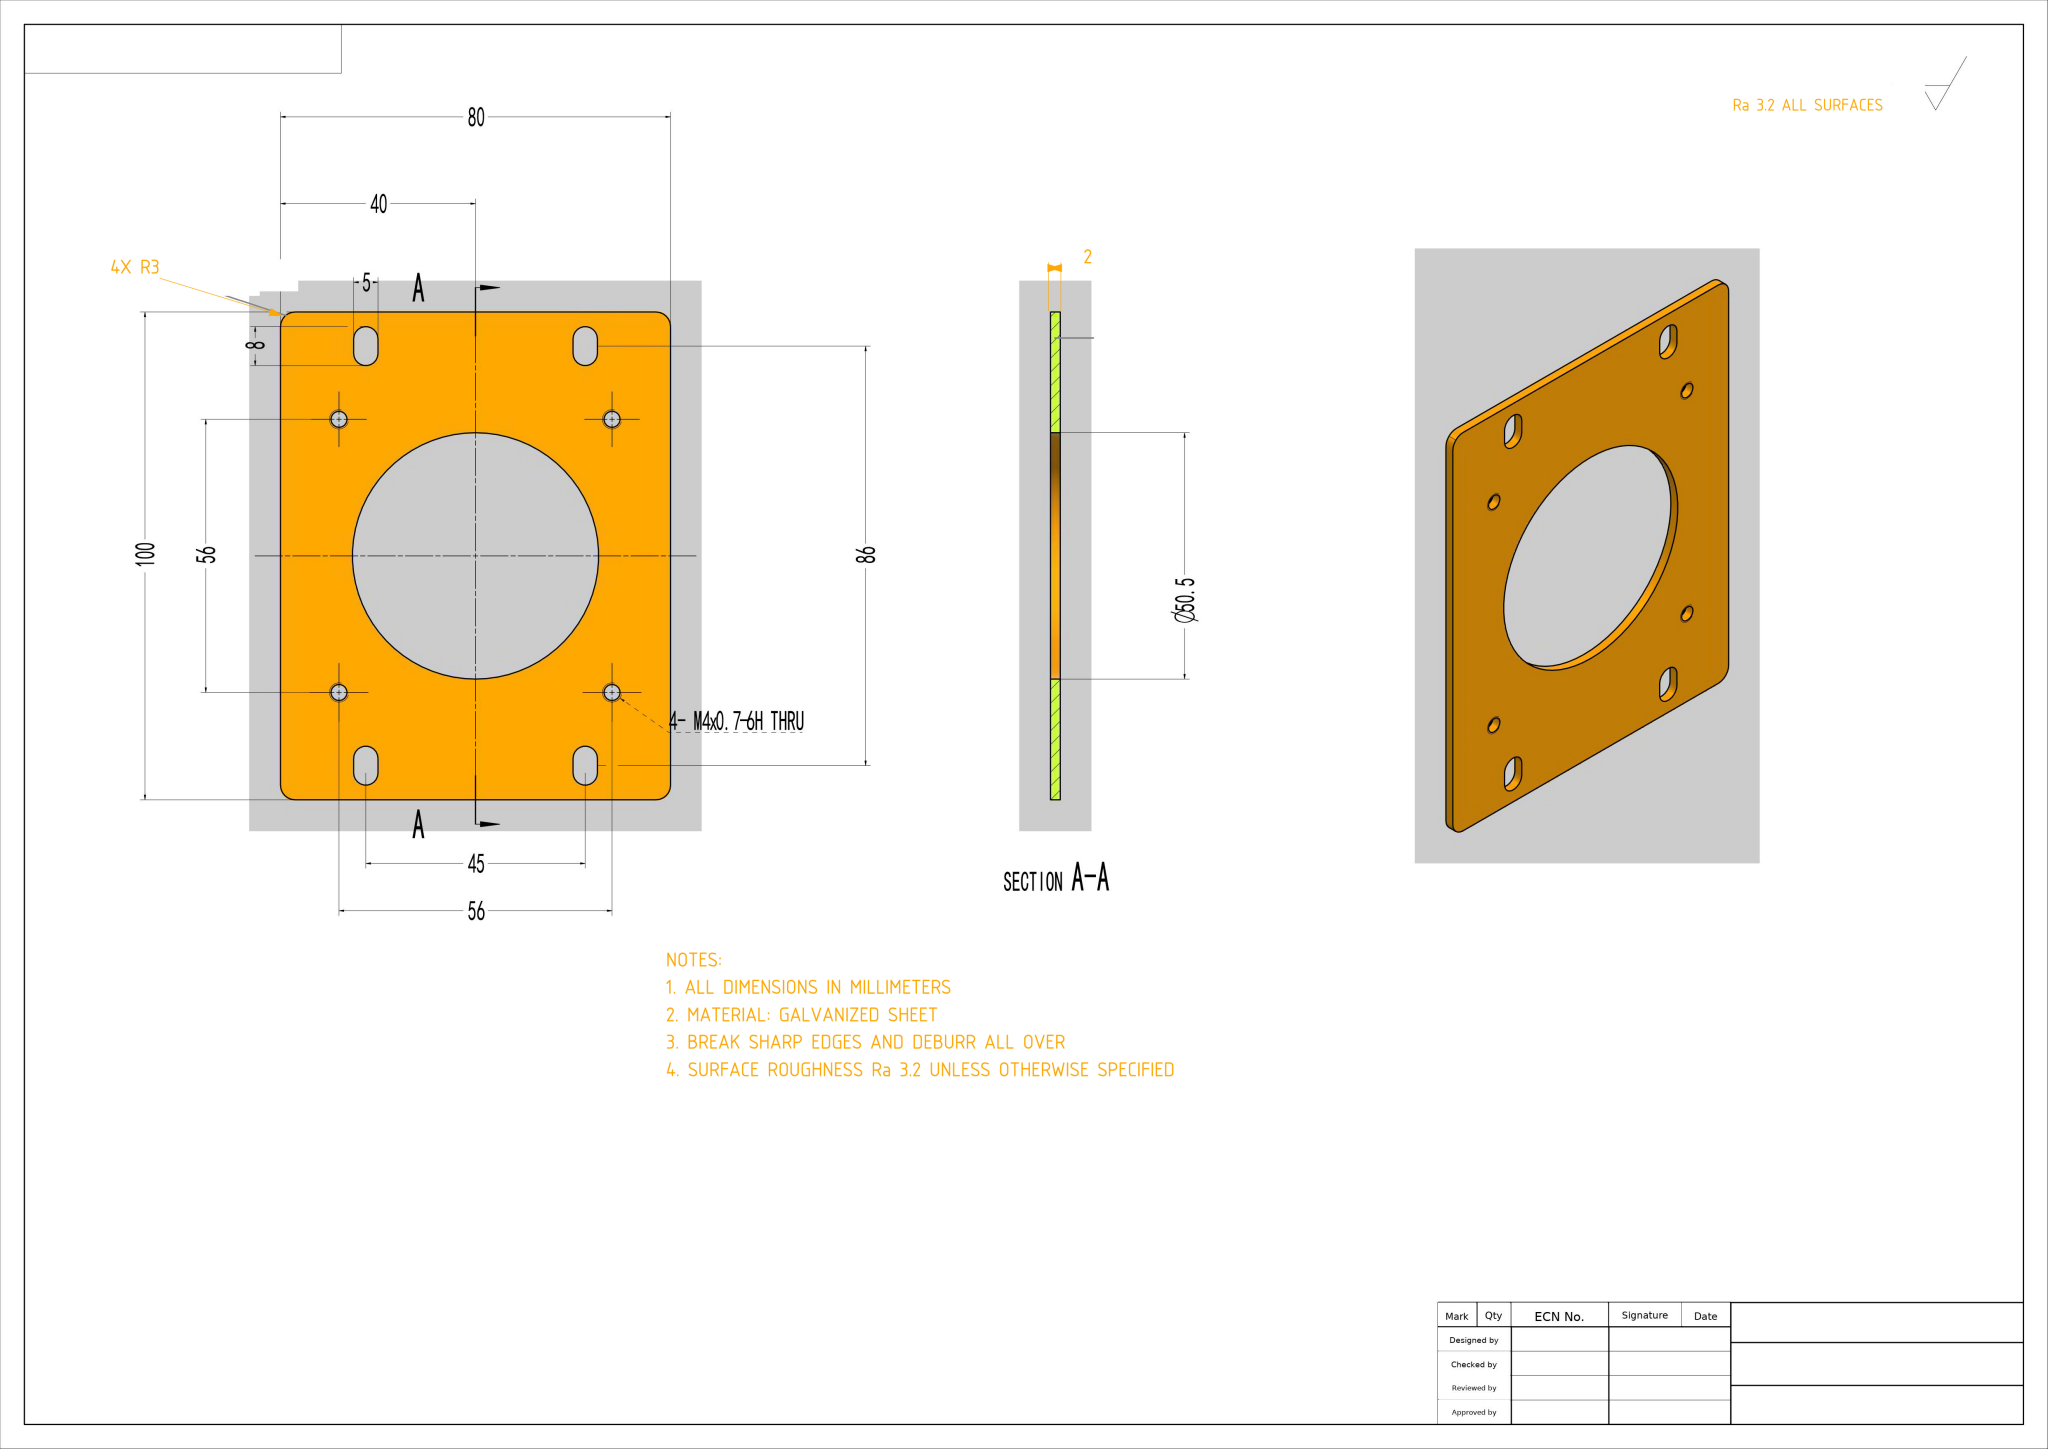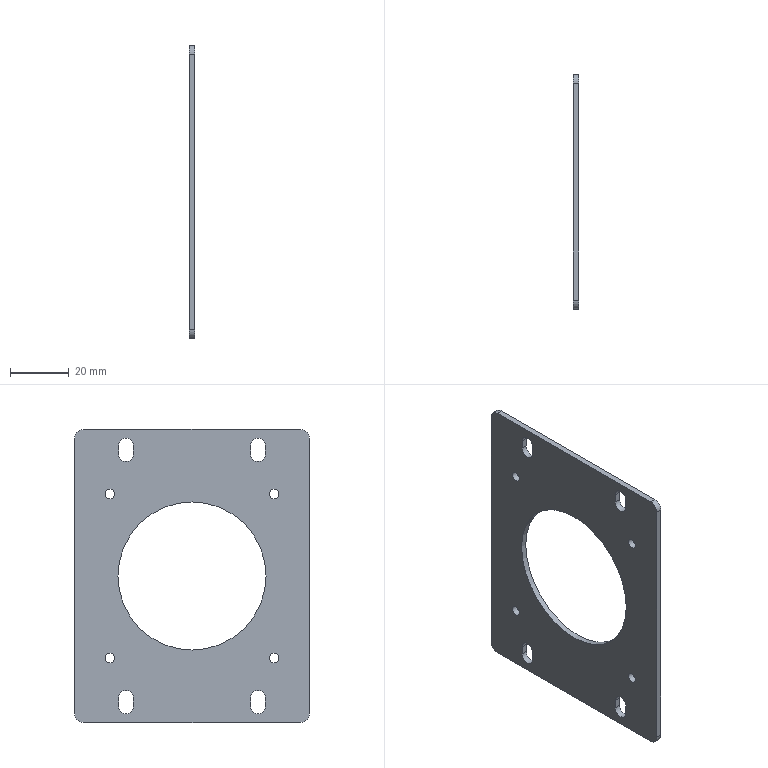Part | NX | mm | 1 solid | 31 faces | box 2 x 80 x 100 mm | volume 11633 mm3 | cylinder 17 | plane 14 | commonest cylinder face diameters 5 x8 3.3 x4 6 x4 50.5 x1
STEP:
#1=CARTESIAN_POINT('',(0.,0.,0.));
#2=DIRECTION('',(0.,0.,1.));
#3=DIRECTION('',(1.,0.,0.));
#4=AXIS2_PLACEMENT_3D('',#1,#2,#3);
#5=(LENGTH_UNIT()NAMED_UNIT(*)SI_UNIT(.MILLI.,.METRE.));
#6=UNCERTAINTY_MEASURE_WITH_UNIT(LENGTH_MEASURE(0.00002),#5,'','');
#7=(NAMED_UNIT(*)PLANE_ANGLE_UNIT()SI_UNIT($,.RADIAN.));
#8=PLANE_ANGLE_MEASURE_WITH_UNIT(PLANE_ANGLE_MEASURE(0.01745),#7);
#9=DIMENSIONAL_EXPONENTS(0.,0.,0.,0.,0.,0.,0.);
#10=(CONVERSION_BASED_UNIT('',#8)NAMED_UNIT(#9)PLANE_ANGLE_UNIT());
#11=(NAMED_UNIT(*)SI_UNIT($,.STERADIAN.)SOLID_ANGLE_UNIT());
#12=(GEOMETRIC_REPRESENTATION_CONTEXT(3)GLOBAL_UNCERTAINTY_ASSIGNED_CONTEXT((#6))GLOBAL_UNIT_ASSIGNED_CONTEXT((#5,#10,#11))REPRESENTATION_CONTEXT('',''));
#13=SHAPE_REPRESENTATION('',(#4),#12);
#14=CARTESIAN_POINT('',(0.,-40.,47.));
#15=VERTEX_POINT('',#14);
#16=CARTESIAN_POINT('',(0.,-40.,-47.));
#17=VERTEX_POINT('',#16);
#18=CARTESIAN_POINT('',(0.,-40.,50.));
#19=DIRECTION('',(0.,0.,-1.));
#20=VECTOR('',#19,1.);
#21=LINE('',#18,#20);
#22=EDGE_CURVE('',#15,#17,#21,.T.);
#23=ORIENTED_EDGE('',*,*,#22,.T.);
#24=CARTESIAN_POINT('',(2.,-40.,-47.));
#25=VERTEX_POINT('',#24);
#26=CARTESIAN_POINT('',(2.,-40.,-47.));
#27=DIRECTION('',(1.,0.,0.));
#28=VECTOR('',#27,1.);
#29=LINE('',#26,#28);
#30=EDGE_CURVE('',#17,#25,#29,.T.);
#31=ORIENTED_EDGE('',*,*,#30,.T.);
#32=CARTESIAN_POINT('',(2.,-40.,47.));
#33=VERTEX_POINT('',#32);
#34=CARTESIAN_POINT('',(2.,-40.,50.));
#35=DIRECTION('',(0.,0.,-1.));
#36=VECTOR('',#35,1.);
#37=LINE('',#34,#36);
#38=EDGE_CURVE('',#33,#25,#37,.T.);
#39=ORIENTED_EDGE('',*,*,#38,.F.);
#40=CARTESIAN_POINT('',(2.,-40.,47.));
#41=DIRECTION('',(-1.,0.,0.));
#42=VECTOR('',#41,1.);
#43=LINE('',#40,#42);
#44=EDGE_CURVE('',#33,#15,#43,.T.);
#45=ORIENTED_EDGE('',*,*,#44,.T.);
#46=EDGE_LOOP('',(#23,#31,#39,#45));
#47=FACE_OUTER_BOUND('',#46,.T.);
#48=CARTESIAN_POINT('',(2.,-40.,50.));
#49=DIRECTION('',(0.,1.,0.));
#50=DIRECTION('',(0.,-0.,1.));
#51=AXIS2_PLACEMENT_3D('',#48,#49,#50);
#52=PLANE('',#51);
#53=ADVANCED_FACE('',(#47),#52,.F.);
#54=CARTESIAN_POINT('',(0.,-37.,-50.));
#55=VERTEX_POINT('',#54);
#56=CARTESIAN_POINT('',(0.,37.,-50.));
#57=VERTEX_POINT('',#56);
#58=CARTESIAN_POINT('',(0.,-40.,-50.));
#59=DIRECTION('',(0.,1.,0.));
#60=VECTOR('',#59,1.);
#61=LINE('',#58,#60);
#62=EDGE_CURVE('',#55,#57,#61,.T.);
#63=ORIENTED_EDGE('',*,*,#62,.T.);
#64=CARTESIAN_POINT('',(2.,37.,-50.));
#65=VERTEX_POINT('',#64);
#66=CARTESIAN_POINT('',(2.,37.,-50.));
#67=DIRECTION('',(1.,0.,0.));
#68=VECTOR('',#67,1.);
#69=LINE('',#66,#68);
#70=EDGE_CURVE('',#57,#65,#69,.T.);
#71=ORIENTED_EDGE('',*,*,#70,.T.);
#72=CARTESIAN_POINT('',(2.,-37.,-50.));
#73=VERTEX_POINT('',#72);
#74=CARTESIAN_POINT('',(2.,-40.,-50.));
#75=DIRECTION('',(0.,1.,0.));
#76=VECTOR('',#75,1.);
#77=LINE('',#74,#76);
#78=EDGE_CURVE('',#73,#65,#77,.T.);
#79=ORIENTED_EDGE('',*,*,#78,.F.);
#80=CARTESIAN_POINT('',(2.,-37.,-50.));
#81=DIRECTION('',(-1.,0.,0.));
#82=VECTOR('',#81,1.);
#83=LINE('',#80,#82);
#84=EDGE_CURVE('',#73,#55,#83,.T.);
#85=ORIENTED_EDGE('',*,*,#84,.T.);
#86=EDGE_LOOP('',(#63,#71,#79,#85));
#87=FACE_OUTER_BOUND('',#86,.T.);
#88=CARTESIAN_POINT('',(2.,-40.,-50.));
#89=DIRECTION('',(0.,-0.,1.));
#90=DIRECTION('',(0.,-1.,-0.));
#91=AXIS2_PLACEMENT_3D('',#88,#89,#90);
#92=PLANE('',#91);
#93=ADVANCED_FACE('',(#87),#92,.F.);
#94=CARTESIAN_POINT('',(2.,40.,-47.));
#95=VERTEX_POINT('',#94);
#96=CARTESIAN_POINT('',(2.,40.,47.));
#97=VERTEX_POINT('',#96);
#98=CARTESIAN_POINT('',(2.,40.,-50.));
#99=DIRECTION('',(0.,-0.,1.));
#100=VECTOR('',#99,1.);
#101=LINE('',#98,#100);
#102=EDGE_CURVE('',#95,#97,#101,.T.);
#103=ORIENTED_EDGE('',*,*,#102,.F.);
#104=CARTESIAN_POINT('',(0.,40.,-47.));
#105=VERTEX_POINT('',#104);
#106=CARTESIAN_POINT('',(2.,40.,-47.));
#107=DIRECTION('',(-1.,0.,0.));
#108=VECTOR('',#107,1.);
#109=LINE('',#106,#108);
#110=EDGE_CURVE('',#95,#105,#109,.T.);
#111=ORIENTED_EDGE('',*,*,#110,.T.);
#112=CARTESIAN_POINT('',(0.,40.,47.));
#113=VERTEX_POINT('',#112);
#114=CARTESIAN_POINT('',(0.,40.,-50.));
#115=DIRECTION('',(0.,-0.,1.));
#116=VECTOR('',#115,1.);
#117=LINE('',#114,#116);
#118=EDGE_CURVE('',#105,#113,#117,.T.);
#119=ORIENTED_EDGE('',*,*,#118,.T.);
#120=CARTESIAN_POINT('',(2.,40.,47.));
#121=DIRECTION('',(1.,0.,0.));
#122=VECTOR('',#121,1.);
#123=LINE('',#120,#122);
#124=EDGE_CURVE('',#113,#97,#123,.T.);
#125=ORIENTED_EDGE('',*,*,#124,.T.);
#126=EDGE_LOOP('',(#103,#111,#119,#125));
#127=FACE_OUTER_BOUND('',#126,.T.);
#128=CARTESIAN_POINT('',(2.,40.,-50.));
#129=DIRECTION('',(0.,-1.,-0.));
#130=DIRECTION('',(0.,0.,-1.));
#131=AXIS2_PLACEMENT_3D('',#128,#129,#130);
#132=PLANE('',#131);
#133=ADVANCED_FACE('',(#127),#132,.F.);
#134=CARTESIAN_POINT('',(0.,37.,50.));
#135=VERTEX_POINT('',#134);
#136=CARTESIAN_POINT('',(0.,-37.,50.));
#137=VERTEX_POINT('',#136);
#138=CARTESIAN_POINT('',(0.,40.,50.));
#139=DIRECTION('',(0.,-1.,-0.));
#140=VECTOR('',#139,1.);
#141=LINE('',#138,#140);
#142=EDGE_CURVE('',#135,#137,#141,.T.);
#143=ORIENTED_EDGE('',*,*,#142,.T.);
#144=CARTESIAN_POINT('',(2.,-37.,50.));
#145=VERTEX_POINT('',#144);
#146=CARTESIAN_POINT('',(2.,-37.,50.));
#147=DIRECTION('',(1.,0.,0.));
#148=VECTOR('',#147,1.);
#149=LINE('',#146,#148);
#150=EDGE_CURVE('',#137,#145,#149,.T.);
#151=ORIENTED_EDGE('',*,*,#150,.T.);
#152=CARTESIAN_POINT('',(2.,37.,50.));
#153=VERTEX_POINT('',#152);
#154=CARTESIAN_POINT('',(2.,40.,50.));
#155=DIRECTION('',(0.,-1.,-0.));
#156=VECTOR('',#155,1.);
#157=LINE('',#154,#156);
#158=EDGE_CURVE('',#153,#145,#157,.T.);
#159=ORIENTED_EDGE('',*,*,#158,.F.);
#160=CARTESIAN_POINT('',(2.,37.,50.));
#161=DIRECTION('',(-1.,0.,0.));
#162=VECTOR('',#161,1.);
#163=LINE('',#160,#162);
#164=EDGE_CURVE('',#153,#135,#163,.T.);
#165=ORIENTED_EDGE('',*,*,#164,.T.);
#166=EDGE_LOOP('',(#143,#151,#159,#165));
#167=FACE_OUTER_BOUND('',#166,.T.);
#168=CARTESIAN_POINT('',(2.,40.,50.));
#169=DIRECTION('',(0.,0.,-1.));
#170=DIRECTION('',(0.,1.,0.));
#171=AXIS2_PLACEMENT_3D('',#168,#169,#170);
#172=PLANE('',#171);
#173=ADVANCED_FACE('',(#167),#172,.F.);
#174=CARTESIAN_POINT('',(2.,-25.,-41.5));
#175=VERTEX_POINT('',#174);
#176=CARTESIAN_POINT('',(2.,-25.,-44.5));
#177=VERTEX_POINT('',#176);
#178=CARTESIAN_POINT('',(2.,-25.,0.));
#179=DIRECTION('',(0.,0.,-1.));
#180=VECTOR('',#179,1.);
#181=LINE('',#178,#180);
#182=EDGE_CURVE('',#175,#177,#181,.T.);
#183=ORIENTED_EDGE('',*,*,#182,.F.);
#184=CARTESIAN_POINT('',(2.,-20.,-41.5));
#185=VERTEX_POINT('',#184);
#186=CARTESIAN_POINT('',(2.,-22.5,-41.5));
#187=DIRECTION('',(1.,0.,0.));
#188=DIRECTION('',(0.,0.,-1.));
#189=AXIS2_PLACEMENT_3D('',#186,#187,#188);
#190=CIRCLE('',#189,2.5);
#191=EDGE_CURVE('',#185,#175,#190,.T.);
#192=ORIENTED_EDGE('',*,*,#191,.F.);
#193=CARTESIAN_POINT('',(2.,-20.,-44.5));
#194=VERTEX_POINT('',#193);
#195=CARTESIAN_POINT('',(2.,-20.,0.));
#196=DIRECTION('',(0.,0.,1.));
#197=VECTOR('',#196,1.);
#198=LINE('',#195,#197);
#199=EDGE_CURVE('',#194,#185,#198,.T.);
#200=ORIENTED_EDGE('',*,*,#199,.F.);
#201=CARTESIAN_POINT('',(2.,-22.5,-44.5));
#202=DIRECTION('',(1.,0.,0.));
#203=DIRECTION('',(0.,0.,-1.));
#204=AXIS2_PLACEMENT_3D('',#201,#202,#203);
#205=CIRCLE('',#204,2.5);
#206=EDGE_CURVE('',#177,#194,#205,.T.);
#207=ORIENTED_EDGE('',*,*,#206,.F.);
#208=EDGE_LOOP('',(#183,#192,#200,#207));
#209=FACE_BOUND('',#208,.T.);
#210=CARTESIAN_POINT('',(2.,20.,-41.5));
#211=VERTEX_POINT('',#210);
#212=CARTESIAN_POINT('',(2.,20.,-44.5));
#213=VERTEX_POINT('',#212);
#214=CARTESIAN_POINT('',(2.,20.,0.));
#215=DIRECTION('',(0.,0.,-1.));
#216=VECTOR('',#215,1.);
#217=LINE('',#214,#216);
#218=EDGE_CURVE('',#211,#213,#217,.T.);
#219=ORIENTED_EDGE('',*,*,#218,.F.);
#220=CARTESIAN_POINT('',(2.,25.,-41.5));
#221=VERTEX_POINT('',#220);
#222=CARTESIAN_POINT('',(2.,22.5,-41.5));
#223=DIRECTION('',(1.,0.,0.));
#224=DIRECTION('',(0.,0.,-1.));
#225=AXIS2_PLACEMENT_3D('',#222,#223,#224);
#226=CIRCLE('',#225,2.5);
#227=EDGE_CURVE('',#221,#211,#226,.T.);
#228=ORIENTED_EDGE('',*,*,#227,.F.);
#229=CARTESIAN_POINT('',(2.,25.,-44.5));
#230=VERTEX_POINT('',#229);
#231=CARTESIAN_POINT('',(2.,25.,0.));
#232=DIRECTION('',(0.,0.,1.));
#233=VECTOR('',#232,1.);
#234=LINE('',#231,#233);
#235=EDGE_CURVE('',#230,#221,#234,.T.);
#236=ORIENTED_EDGE('',*,*,#235,.F.);
#237=CARTESIAN_POINT('',(2.,22.5,-44.5));
#238=DIRECTION('',(1.,0.,0.));
#239=DIRECTION('',(0.,0.,-1.));
#240=AXIS2_PLACEMENT_3D('',#237,#238,#239);
#241=CIRCLE('',#240,2.5);
#242=EDGE_CURVE('',#213,#230,#241,.T.);
#243=ORIENTED_EDGE('',*,*,#242,.F.);
#244=EDGE_LOOP('',(#219,#228,#236,#243));
#245=FACE_BOUND('',#244,.T.);
#246=CARTESIAN_POINT('',(2.,-25.,44.5));
#247=VERTEX_POINT('',#246);
#248=CARTESIAN_POINT('',(2.,-25.,41.5));
#249=VERTEX_POINT('',#248);
#250=CARTESIAN_POINT('',(2.,-25.,0.));
#251=DIRECTION('',(0.,0.,-1.));
#252=VECTOR('',#251,1.);
#253=LINE('',#250,#252);
#254=EDGE_CURVE('',#247,#249,#253,.T.);
#255=ORIENTED_EDGE('',*,*,#254,.F.);
#256=CARTESIAN_POINT('',(2.,-20.,44.5));
#257=VERTEX_POINT('',#256);
#258=CARTESIAN_POINT('',(2.,-22.5,44.5));
#259=DIRECTION('',(1.,0.,0.));
#260=DIRECTION('',(0.,0.,-1.));
#261=AXIS2_PLACEMENT_3D('',#258,#259,#260);
#262=CIRCLE('',#261,2.5);
#263=EDGE_CURVE('',#257,#247,#262,.T.);
#264=ORIENTED_EDGE('',*,*,#263,.F.);
#265=CARTESIAN_POINT('',(2.,-20.,41.5));
#266=VERTEX_POINT('',#265);
#267=CARTESIAN_POINT('',(2.,-20.,0.));
#268=DIRECTION('',(0.,0.,1.));
#269=VECTOR('',#268,1.);
#270=LINE('',#267,#269);
#271=EDGE_CURVE('',#266,#257,#270,.T.);
#272=ORIENTED_EDGE('',*,*,#271,.F.);
#273=CARTESIAN_POINT('',(2.,-22.5,41.5));
#274=DIRECTION('',(1.,0.,0.));
#275=DIRECTION('',(0.,0.,-1.));
#276=AXIS2_PLACEMENT_3D('',#273,#274,#275);
#277=CIRCLE('',#276,2.5);
#278=EDGE_CURVE('',#249,#266,#277,.T.);
#279=ORIENTED_EDGE('',*,*,#278,.F.);
#280=EDGE_LOOP('',(#255,#264,#272,#279));
#281=FACE_BOUND('',#280,.T.);
#282=CARTESIAN_POINT('',(2.,20.,44.5));
#283=VERTEX_POINT('',#282);
#284=CARTESIAN_POINT('',(2.,20.,41.5));
#285=VERTEX_POINT('',#284);
#286=CARTESIAN_POINT('',(2.,20.,0.));
#287=DIRECTION('',(0.,0.,-1.));
#288=VECTOR('',#287,1.);
#289=LINE('',#286,#288);
#290=EDGE_CURVE('',#283,#285,#289,.T.);
#291=ORIENTED_EDGE('',*,*,#290,.F.);
#292=CARTESIAN_POINT('',(2.,25.,44.5));
#293=VERTEX_POINT('',#292);
#294=CARTESIAN_POINT('',(2.,22.5,44.5));
#295=DIRECTION('',(1.,0.,0.));
#296=DIRECTION('',(0.,0.,-1.));
#297=AXIS2_PLACEMENT_3D('',#294,#295,#296);
#298=CIRCLE('',#297,2.5);
#299=EDGE_CURVE('',#293,#283,#298,.T.);
#300=ORIENTED_EDGE('',*,*,#299,.F.);
#301=CARTESIAN_POINT('',(2.,25.,41.5));
#302=VERTEX_POINT('',#301);
#303=CARTESIAN_POINT('',(2.,25.,0.));
#304=DIRECTION('',(0.,0.,1.));
#305=VECTOR('',#304,1.);
#306=LINE('',#303,#305);
#307=EDGE_CURVE('',#302,#293,#306,.T.);
#308=ORIENTED_EDGE('',*,*,#307,.F.);
#309=CARTESIAN_POINT('',(2.,22.5,41.5));
#310=DIRECTION('',(1.,0.,0.));
#311=DIRECTION('',(0.,0.,-1.));
#312=AXIS2_PLACEMENT_3D('',#309,#310,#311);
#313=CIRCLE('',#312,2.5);
#314=EDGE_CURVE('',#285,#302,#313,.T.);
#315=ORIENTED_EDGE('',*,*,#314,.F.);
#316=EDGE_LOOP('',(#291,#300,#308,#315));
#317=FACE_BOUND('',#316,.T.);
#318=CARTESIAN_POINT('',(2.,28.,26.35));
#319=VERTEX_POINT('',#318);
#320=CARTESIAN_POINT('',(2.,28.,28.));
#321=DIRECTION('',(1.,0.,0.));
#322=DIRECTION('',(0.,0.,-1.));
#323=AXIS2_PLACEMENT_3D('',#320,#321,#322);
#324=CIRCLE('',#323,1.65);
#325=EDGE_CURVE('',#319,#319,#324,.T.);
#326=ORIENTED_EDGE('',*,*,#325,.F.);
#327=EDGE_LOOP('',(#326));
#328=FACE_BOUND('',#327,.T.);
#329=CARTESIAN_POINT('',(2.,28.,-29.65));
#330=VERTEX_POINT('',#329);
#331=CARTESIAN_POINT('',(2.,28.,-28.));
#332=DIRECTION('',(1.,0.,0.));
#333=DIRECTION('',(0.,0.,-1.));
#334=AXIS2_PLACEMENT_3D('',#331,#332,#333);
#335=CIRCLE('',#334,1.65);
#336=EDGE_CURVE('',#330,#330,#335,.T.);
#337=ORIENTED_EDGE('',*,*,#336,.F.);
#338=EDGE_LOOP('',(#337));
#339=FACE_BOUND('',#338,.T.);
#340=CARTESIAN_POINT('',(2.,-28.,26.35));
#341=VERTEX_POINT('',#340);
#342=CARTESIAN_POINT('',(2.,-28.,28.));
#343=DIRECTION('',(1.,0.,0.));
#344=DIRECTION('',(0.,0.,-1.));
#345=AXIS2_PLACEMENT_3D('',#342,#343,#344);
#346=CIRCLE('',#345,1.65);
#347=EDGE_CURVE('',#341,#341,#346,.T.);
#348=ORIENTED_EDGE('',*,*,#347,.F.);
#349=EDGE_LOOP('',(#348));
#350=FACE_BOUND('',#349,.T.);
#351=CARTESIAN_POINT('',(2.,-28.,-29.65));
#352=VERTEX_POINT('',#351);
#353=CARTESIAN_POINT('',(2.,-28.,-28.));
#354=DIRECTION('',(1.,0.,0.));
#355=DIRECTION('',(0.,0.,-1.));
#356=AXIS2_PLACEMENT_3D('',#353,#354,#355);
#357=CIRCLE('',#356,1.65);
#358=EDGE_CURVE('',#352,#352,#357,.T.);
#359=ORIENTED_EDGE('',*,*,#358,.F.);
#360=EDGE_LOOP('',(#359));
#361=FACE_BOUND('',#360,.T.);
#362=CARTESIAN_POINT('',(2.,0.,-25.25));
#363=VERTEX_POINT('',#362);
#364=CARTESIAN_POINT('',(2.,0.,0.));
#365=DIRECTION('',(1.,0.,0.));
#366=DIRECTION('',(0.,0.,-1.));
#367=AXIS2_PLACEMENT_3D('',#364,#365,#366);
#368=CIRCLE('',#367,25.25);
#369=EDGE_CURVE('',#363,#363,#368,.T.);
#370=ORIENTED_EDGE('',*,*,#369,.F.);
#371=EDGE_LOOP('',(#370));
#372=FACE_BOUND('',#371,.T.);
#373=ORIENTED_EDGE('',*,*,#78,.T.);
#374=CARTESIAN_POINT('',(2.,37.,-47.));
#375=DIRECTION('',(1.,0.,0.));
#376=DIRECTION('',(0.,0.,-1.));
#377=AXIS2_PLACEMENT_3D('',#374,#375,#376);
#378=CIRCLE('',#377,3.);
#379=EDGE_CURVE('',#65,#95,#378,.T.);
#380=ORIENTED_EDGE('',*,*,#379,.T.);
#381=ORIENTED_EDGE('',*,*,#102,.T.);
#382=CARTESIAN_POINT('',(2.,37.,47.));
#383=DIRECTION('',(1.,0.,0.));
#384=DIRECTION('',(0.,0.,-1.));
#385=AXIS2_PLACEMENT_3D('',#382,#383,#384);
#386=CIRCLE('',#385,3.);
#387=EDGE_CURVE('',#97,#153,#386,.T.);
#388=ORIENTED_EDGE('',*,*,#387,.T.);
#389=ORIENTED_EDGE('',*,*,#158,.T.);
#390=CARTESIAN_POINT('',(2.,-37.,47.));
#391=DIRECTION('',(1.,0.,0.));
#392=DIRECTION('',(0.,0.,-1.));
#393=AXIS2_PLACEMENT_3D('',#390,#391,#392);
#394=CIRCLE('',#393,3.);
#395=EDGE_CURVE('',#145,#33,#394,.T.);
#396=ORIENTED_EDGE('',*,*,#395,.T.);
#397=ORIENTED_EDGE('',*,*,#38,.T.);
#398=CARTESIAN_POINT('',(2.,-37.,-47.));
#399=DIRECTION('',(1.,0.,0.));
#400=DIRECTION('',(0.,0.,-1.));
#401=AXIS2_PLACEMENT_3D('',#398,#399,#400);
#402=CIRCLE('',#401,3.);
#403=EDGE_CURVE('',#25,#73,#402,.T.);
#404=ORIENTED_EDGE('',*,*,#403,.T.);
#405=EDGE_LOOP('',(#373,#380,#381,#388,#389,#396,#397,#404));
#406=FACE_BOUND('',#405,.T.);
#407=CARTESIAN_POINT('',(2.,0.,0.));
#408=DIRECTION('',(1.,0.,0.));
#409=DIRECTION('',(0.,0.,-1.));
#410=AXIS2_PLACEMENT_3D('',#407,#408,#409);
#411=PLANE('',#410);
#412=ADVANCED_FACE('',(#209,#245,#281,#317,#328,#339,#350,#361,#372,#406),#411,.T.);
#413=CARTESIAN_POINT('',(0.,-25.,-41.5));
#414=VERTEX_POINT('',#413);
#415=CARTESIAN_POINT('',(0.,-20.,-41.5));
#416=VERTEX_POINT('',#415);
#417=CARTESIAN_POINT('',(0.,-22.5,-41.5));
#418=DIRECTION('',(-1.,0.,0.));
#419=DIRECTION('',(0.,-1.,0.));
#420=AXIS2_PLACEMENT_3D('',#417,#418,#419);
#421=CIRCLE('',#420,2.5);
#422=EDGE_CURVE('',#414,#416,#421,.T.);
#423=ORIENTED_EDGE('',*,*,#422,.F.);
#424=CARTESIAN_POINT('',(0.,-25.,-44.5));
#425=VERTEX_POINT('',#424);
#426=CARTESIAN_POINT('',(0.,-25.,-44.5));
#427=DIRECTION('',(0.,0.,1.));
#428=VECTOR('',#427,1.);
#429=LINE('',#426,#428);
#430=EDGE_CURVE('',#425,#414,#429,.T.);
#431=ORIENTED_EDGE('',*,*,#430,.F.);
#432=CARTESIAN_POINT('',(0.,-20.,-44.5));
#433=VERTEX_POINT('',#432);
#434=CARTESIAN_POINT('',(0.,-22.5,-44.5));
#435=DIRECTION('',(-1.,0.,0.));
#436=DIRECTION('',(0.,-1.,0.));
#437=AXIS2_PLACEMENT_3D('',#434,#435,#436);
#438=CIRCLE('',#437,2.5);
#439=EDGE_CURVE('',#433,#425,#438,.T.);
#440=ORIENTED_EDGE('',*,*,#439,.F.);
#441=CARTESIAN_POINT('',(0.,-20.,-41.5));
#442=DIRECTION('',(0.,0.,-1.));
#443=VECTOR('',#442,1.);
#444=LINE('',#441,#443);
#445=EDGE_CURVE('',#416,#433,#444,.T.);
#446=ORIENTED_EDGE('',*,*,#445,.F.);
#447=EDGE_LOOP('',(#423,#431,#440,#446));
#448=FACE_BOUND('',#447,.T.);
#449=CARTESIAN_POINT('',(0.,20.,-41.5));
#450=VERTEX_POINT('',#449);
#451=CARTESIAN_POINT('',(0.,25.,-41.5));
#452=VERTEX_POINT('',#451);
#453=CARTESIAN_POINT('',(0.,22.5,-41.5));
#454=DIRECTION('',(-1.,0.,0.));
#455=DIRECTION('',(0.,-1.,0.));
#456=AXIS2_PLACEMENT_3D('',#453,#454,#455);
#457=CIRCLE('',#456,2.5);
#458=EDGE_CURVE('',#450,#452,#457,.T.);
#459=ORIENTED_EDGE('',*,*,#458,.F.);
#460=CARTESIAN_POINT('',(0.,20.,-44.5));
#461=VERTEX_POINT('',#460);
#462=CARTESIAN_POINT('',(0.,20.,-44.5));
#463=DIRECTION('',(0.,0.,1.));
#464=VECTOR('',#463,1.);
#465=LINE('',#462,#464);
#466=EDGE_CURVE('',#461,#450,#465,.T.);
#467=ORIENTED_EDGE('',*,*,#466,.F.);
#468=CARTESIAN_POINT('',(0.,25.,-44.5));
#469=VERTEX_POINT('',#468);
#470=CARTESIAN_POINT('',(0.,22.5,-44.5));
#471=DIRECTION('',(-1.,0.,0.));
#472=DIRECTION('',(0.,-1.,0.));
#473=AXIS2_PLACEMENT_3D('',#470,#471,#472);
#474=CIRCLE('',#473,2.5);
#475=EDGE_CURVE('',#469,#461,#474,.T.);
#476=ORIENTED_EDGE('',*,*,#475,.F.);
#477=CARTESIAN_POINT('',(0.,25.,-41.5));
#478=DIRECTION('',(0.,0.,-1.));
#479=VECTOR('',#478,1.);
#480=LINE('',#477,#479);
#481=EDGE_CURVE('',#452,#469,#480,.T.);
#482=ORIENTED_EDGE('',*,*,#481,.F.);
#483=EDGE_LOOP('',(#459,#467,#476,#482));
#484=FACE_BOUND('',#483,.T.);
#485=CARTESIAN_POINT('',(0.,-25.,44.5));
#486=VERTEX_POINT('',#485);
#487=CARTESIAN_POINT('',(0.,-20.,44.5));
#488=VERTEX_POINT('',#487);
#489=CARTESIAN_POINT('',(0.,-22.5,44.5));
#490=DIRECTION('',(-1.,0.,0.));
#491=DIRECTION('',(0.,-1.,0.));
#492=AXIS2_PLACEMENT_3D('',#489,#490,#491);
#493=CIRCLE('',#492,2.5);
#494=EDGE_CURVE('',#486,#488,#493,.T.);
#495=ORIENTED_EDGE('',*,*,#494,.F.);
#496=CARTESIAN_POINT('',(0.,-25.,41.5));
#497=VERTEX_POINT('',#496);
#498=CARTESIAN_POINT('',(0.,-25.,41.5));
#499=DIRECTION('',(0.,0.,1.));
#500=VECTOR('',#499,1.);
#501=LINE('',#498,#500);
#502=EDGE_CURVE('',#497,#486,#501,.T.);
#503=ORIENTED_EDGE('',*,*,#502,.F.);
#504=CARTESIAN_POINT('',(0.,-20.,41.5));
#505=VERTEX_POINT('',#504);
#506=CARTESIAN_POINT('',(0.,-22.5,41.5));
#507=DIRECTION('',(-1.,0.,0.));
#508=DIRECTION('',(0.,-1.,0.));
#509=AXIS2_PLACEMENT_3D('',#506,#507,#508);
#510=CIRCLE('',#509,2.5);
#511=EDGE_CURVE('',#505,#497,#510,.T.);
#512=ORIENTED_EDGE('',*,*,#511,.F.);
#513=CARTESIAN_POINT('',(0.,-20.,44.5));
#514=DIRECTION('',(0.,0.,-1.));
#515=VECTOR('',#514,1.);
#516=LINE('',#513,#515);
#517=EDGE_CURVE('',#488,#505,#516,.T.);
#518=ORIENTED_EDGE('',*,*,#517,.F.);
#519=EDGE_LOOP('',(#495,#503,#512,#518));
#520=FACE_BOUND('',#519,.T.);
#521=CARTESIAN_POINT('',(0.,20.,44.5));
#522=VERTEX_POINT('',#521);
#523=CARTESIAN_POINT('',(0.,25.,44.5));
#524=VERTEX_POINT('',#523);
#525=CARTESIAN_POINT('',(0.,22.5,44.5));
#526=DIRECTION('',(-1.,0.,0.));
#527=DIRECTION('',(0.,-1.,0.));
#528=AXIS2_PLACEMENT_3D('',#525,#526,#527);
#529=CIRCLE('',#528,2.5);
#530=EDGE_CURVE('',#522,#524,#529,.T.);
#531=ORIENTED_EDGE('',*,*,#530,.F.);
#532=CARTESIAN_POINT('',(0.,20.,41.5));
#533=VERTEX_POINT('',#532);
#534=CARTESIAN_POINT('',(0.,20.,41.5));
#535=DIRECTION('',(0.,0.,1.));
#536=VECTOR('',#535,1.);
#537=LINE('',#534,#536);
#538=EDGE_CURVE('',#533,#522,#537,.T.);
#539=ORIENTED_EDGE('',*,*,#538,.F.);
#540=CARTESIAN_POINT('',(0.,25.,41.5));
#541=VERTEX_POINT('',#540);
#542=CARTESIAN_POINT('',(0.,22.5,41.5));
#543=DIRECTION('',(-1.,0.,0.));
#544=DIRECTION('',(0.,-1.,0.));
#545=AXIS2_PLACEMENT_3D('',#542,#543,#544);
#546=CIRCLE('',#545,2.5);
#547=EDGE_CURVE('',#541,#533,#546,.T.);
#548=ORIENTED_EDGE('',*,*,#547,.F.);
#549=CARTESIAN_POINT('',(0.,25.,44.5));
#550=DIRECTION('',(0.,0.,-1.));
#551=VECTOR('',#550,1.);
#552=LINE('',#549,#551);
#553=EDGE_CURVE('',#524,#541,#552,.T.);
#554=ORIENTED_EDGE('',*,*,#553,.F.);
#555=EDGE_LOOP('',(#531,#539,#548,#554));
#556=FACE_BOUND('',#555,.T.);
#557=CARTESIAN_POINT('',(0.,28.,26.35));
#558=VERTEX_POINT('',#557);
#559=CARTESIAN_POINT('',(0.,28.,28.));
#560=DIRECTION('',(1.,0.,0.));
#561=DIRECTION('',(0.,0.,-1.));
#562=AXIS2_PLACEMENT_3D('',#559,#560,#561);
#563=CIRCLE('',#562,1.65);
#564=EDGE_CURVE('',#558,#558,#563,.T.);
#565=ORIENTED_EDGE('',*,*,#564,.T.);
#566=EDGE_LOOP('',(#565));
#567=FACE_BOUND('',#566,.T.);
#568=CARTESIAN_POINT('',(0.,28.,-29.65));
#569=VERTEX_POINT('',#568);
#570=CARTESIAN_POINT('',(0.,28.,-28.));
#571=DIRECTION('',(1.,0.,0.));
#572=DIRECTION('',(0.,0.,-1.));
#573=AXIS2_PLACEMENT_3D('',#570,#571,#572);
#574=CIRCLE('',#573,1.65);
#575=EDGE_CURVE('',#569,#569,#574,.T.);
#576=ORIENTED_EDGE('',*,*,#575,.T.);
#577=EDGE_LOOP('',(#576));
#578=FACE_BOUND('',#577,.T.);
#579=CARTESIAN_POINT('',(0.,-28.,26.35));
#580=VERTEX_POINT('',#579);
#581=CARTESIAN_POINT('',(0.,-28.,28.));
#582=DIRECTION('',(1.,0.,0.));
#583=DIRECTION('',(0.,0.,-1.));
#584=AXIS2_PLACEMENT_3D('',#581,#582,#583);
#585=CIRCLE('',#584,1.65);
#586=EDGE_CURVE('',#580,#580,#585,.T.);
#587=ORIENTED_EDGE('',*,*,#586,.T.);
#588=EDGE_LOOP('',(#587));
#589=FACE_BOUND('',#588,.T.);
#590=CARTESIAN_POINT('',(0.,-28.,-29.65));
#591=VERTEX_POINT('',#590);
#592=CARTESIAN_POINT('',(0.,-28.,-28.));
#593=DIRECTION('',(1.,0.,0.));
#594=DIRECTION('',(0.,0.,-1.));
#595=AXIS2_PLACEMENT_3D('',#592,#593,#594);
#596=CIRCLE('',#595,1.65);
#597=EDGE_CURVE('',#591,#591,#596,.T.);
#598=ORIENTED_EDGE('',*,*,#597,.T.);
#599=EDGE_LOOP('',(#598));
#600=FACE_BOUND('',#599,.T.);
#601=CARTESIAN_POINT('',(0.,0.,-25.25));
#602=VERTEX_POINT('',#601);
#603=CARTESIAN_POINT('',(0.,0.,0.));
#604=DIRECTION('',(1.,0.,0.));
#605=DIRECTION('',(0.,0.,-1.));
#606=AXIS2_PLACEMENT_3D('',#603,#604,#605);
#607=CIRCLE('',#606,25.25);
#608=EDGE_CURVE('',#602,#602,#607,.T.);
#609=ORIENTED_EDGE('',*,*,#608,.T.);
#610=EDGE_LOOP('',(#609));
#611=FACE_BOUND('',#610,.T.);
#612=ORIENTED_EDGE('',*,*,#118,.F.);
#613=CARTESIAN_POINT('',(0.,37.,-47.));
#614=DIRECTION('',(-1.,0.,0.));
#615=DIRECTION('',(0.,0.,-1.));
#616=AXIS2_PLACEMENT_3D('',#613,#614,#615);
#617=CIRCLE('',#616,3.);
#618=EDGE_CURVE('',#105,#57,#617,.T.);
#619=ORIENTED_EDGE('',*,*,#618,.T.);
#620=ORIENTED_EDGE('',*,*,#62,.F.);
#621=CARTESIAN_POINT('',(0.,-37.,-47.));
#622=DIRECTION('',(-1.,0.,0.));
#623=DIRECTION('',(0.,0.,-1.));
#624=AXIS2_PLACEMENT_3D('',#621,#622,#623);
#625=CIRCLE('',#624,3.);
#626=EDGE_CURVE('',#55,#17,#625,.T.);
#627=ORIENTED_EDGE('',*,*,#626,.T.);
#628=ORIENTED_EDGE('',*,*,#22,.F.);
#629=CARTESIAN_POINT('',(0.,-37.,47.));
#630=DIRECTION('',(-1.,0.,0.));
#631=DIRECTION('',(0.,0.,-1.));
#632=AXIS2_PLACEMENT_3D('',#629,#630,#631);
#633=CIRCLE('',#632,3.);
#634=EDGE_CURVE('',#15,#137,#633,.T.);
#635=ORIENTED_EDGE('',*,*,#634,.T.);
#636=ORIENTED_EDGE('',*,*,#142,.F.);
#637=CARTESIAN_POINT('',(0.,37.,47.));
#638=DIRECTION('',(-1.,0.,0.));
#639=DIRECTION('',(0.,0.,-1.));
#640=AXIS2_PLACEMENT_3D('',#637,#638,#639);
#641=CIRCLE('',#640,3.);
#642=EDGE_CURVE('',#135,#113,#641,.T.);
#643=ORIENTED_EDGE('',*,*,#642,.T.);
#644=EDGE_LOOP('',(#612,#619,#620,#627,#628,#635,#636,#643));
#645=FACE_BOUND('',#644,.T.);
#646=CARTESIAN_POINT('',(0.,0.,0.));
#647=DIRECTION('',(1.,0.,0.));
#648=DIRECTION('',(0.,0.,-1.));
#649=AXIS2_PLACEMENT_3D('',#646,#647,#648);
#650=PLANE('',#649);
#651=ADVANCED_FACE('',(#448,#484,#520,#556,#567,#578,#589,#600,#611,#645),#650,.F.);
#652=ORIENTED_EDGE('',*,*,#369,.T.);
#653=EDGE_LOOP('',(#652));
#654=FACE_BOUND('',#653,.T.);
#655=ORIENTED_EDGE('',*,*,#608,.F.);
#656=EDGE_LOOP('',(#655));
#657=FACE_BOUND('',#656,.T.);
#658=CARTESIAN_POINT('',(0.,0.,0.));
#659=DIRECTION('',(1.,0.,0.));
#660=DIRECTION('',(0.,0.,-1.));
#661=AXIS2_PLACEMENT_3D('',#658,#659,#660);
#662=CYLINDRICAL_SURFACE('',#661,25.25);
#663=ADVANCED_FACE('',(#654,#657),#662,.F.);
#664=ORIENTED_EDGE('',*,*,#358,.T.);
#665=EDGE_LOOP('',(#664));
#666=FACE_BOUND('',#665,.T.);
#667=ORIENTED_EDGE('',*,*,#597,.F.);
#668=EDGE_LOOP('',(#667));
#669=FACE_BOUND('',#668,.T.);
#670=CARTESIAN_POINT('',(0.,-28.,-28.));
#671=DIRECTION('',(1.,0.,0.));
#672=DIRECTION('',(0.,0.,-1.));
#673=AXIS2_PLACEMENT_3D('',#670,#671,#672);
#674=CYLINDRICAL_SURFACE('',#673,1.65);
#675=ADVANCED_FACE('',(#666,#669),#674,.F.);
#676=ORIENTED_EDGE('',*,*,#347,.T.);
#677=EDGE_LOOP('',(#676));
#678=FACE_BOUND('',#677,.T.);
#679=ORIENTED_EDGE('',*,*,#586,.F.);
#680=EDGE_LOOP('',(#679));
#681=FACE_BOUND('',#680,.T.);
#682=CARTESIAN_POINT('',(0.,-28.,28.));
#683=DIRECTION('',(1.,0.,0.));
#684=DIRECTION('',(0.,0.,-1.));
#685=AXIS2_PLACEMENT_3D('',#682,#683,#684);
#686=CYLINDRICAL_SURFACE('',#685,1.65);
#687=ADVANCED_FACE('',(#678,#681),#686,.F.);
#688=ORIENTED_EDGE('',*,*,#336,.T.);
#689=EDGE_LOOP('',(#688));
#690=FACE_BOUND('',#689,.T.);
#691=ORIENTED_EDGE('',*,*,#575,.F.);
#692=EDGE_LOOP('',(#691));
#693=FACE_BOUND('',#692,.T.);
#694=CARTESIAN_POINT('',(0.,28.,-28.));
#695=DIRECTION('',(1.,0.,0.));
#696=DIRECTION('',(0.,0.,-1.));
#697=AXIS2_PLACEMENT_3D('',#694,#695,#696);
#698=CYLINDRICAL_SURFACE('',#697,1.65);
#699=ADVANCED_FACE('',(#690,#693),#698,.F.);
#700=ORIENTED_EDGE('',*,*,#325,.T.);
#701=EDGE_LOOP('',(#700));
#702=FACE_BOUND('',#701,.T.);
#703=ORIENTED_EDGE('',*,*,#564,.F.);
#704=EDGE_LOOP('',(#703));
#705=FACE_BOUND('',#704,.T.);
#706=CARTESIAN_POINT('',(0.,28.,28.));
#707=DIRECTION('',(1.,0.,0.));
#708=DIRECTION('',(0.,0.,-1.));
#709=AXIS2_PLACEMENT_3D('',#706,#707,#708);
#710=CYLINDRICAL_SURFACE('',#709,1.65);
#711=ADVANCED_FACE('',(#702,#705),#710,.F.);
#712=ORIENTED_EDGE('',*,*,#290,.T.);
#713=CARTESIAN_POINT('',(11.,20.,41.5));
#714=DIRECTION('',(1.,0.,0.));
#715=VECTOR('',#714,1.);
#716=LINE('',#713,#715);
#717=EDGE_CURVE('',#533,#285,#716,.T.);
#718=ORIENTED_EDGE('',*,*,#717,.F.);
#719=ORIENTED_EDGE('',*,*,#538,.T.);
#720=CARTESIAN_POINT('',(11.,20.,44.5));
#721=DIRECTION('',(1.,0.,0.));
#722=VECTOR('',#721,1.);
#723=LINE('',#720,#722);
#724=EDGE_CURVE('',#522,#283,#723,.T.);
#725=ORIENTED_EDGE('',*,*,#724,.T.);
#726=EDGE_LOOP('',(#712,#718,#719,#725));
#727=FACE_OUTER_BOUND('',#726,.T.);
#728=CARTESIAN_POINT('',(11.,20.,41.5));
#729=DIRECTION('',(0.,-1.,0.));
#730=DIRECTION('',(0.,0.,-1.));
#731=AXIS2_PLACEMENT_3D('',#728,#729,#730);
#732=PLANE('',#731);
#733=ADVANCED_FACE('',(#727),#732,.F.);
#734=ORIENTED_EDGE('',*,*,#299,.T.);
#735=ORIENTED_EDGE('',*,*,#724,.F.);
#736=ORIENTED_EDGE('',*,*,#530,.T.);
#737=CARTESIAN_POINT('',(11.,25.,44.5));
#738=DIRECTION('',(1.,0.,0.));
#739=VECTOR('',#738,1.);
#740=LINE('',#737,#739);
#741=EDGE_CURVE('',#524,#293,#740,.T.);
#742=ORIENTED_EDGE('',*,*,#741,.T.);
#743=EDGE_LOOP('',(#734,#735,#736,#742));
#744=FACE_OUTER_BOUND('',#743,.T.);
#745=CARTESIAN_POINT('',(11.,22.5,44.5));
#746=DIRECTION('',(-1.,0.,0.));
#747=DIRECTION('',(0.,0.,1.));
#748=AXIS2_PLACEMENT_3D('',#745,#746,#747);
#749=CYLINDRICAL_SURFACE('',#748,2.5);
#750=ADVANCED_FACE('',(#744),#749,.F.);
#751=ORIENTED_EDGE('',*,*,#307,.T.);
#752=ORIENTED_EDGE('',*,*,#741,.F.);
#753=ORIENTED_EDGE('',*,*,#553,.T.);
#754=CARTESIAN_POINT('',(11.,25.,41.5));
#755=DIRECTION('',(1.,0.,0.));
#756=VECTOR('',#755,1.);
#757=LINE('',#754,#756);
#758=EDGE_CURVE('',#541,#302,#757,.T.);
#759=ORIENTED_EDGE('',*,*,#758,.T.);
#760=EDGE_LOOP('',(#751,#752,#753,#759));
#761=FACE_OUTER_BOUND('',#760,.T.);
#762=CARTESIAN_POINT('',(11.,25.,44.5));
#763=DIRECTION('',(0.,1.,0.));
#764=DIRECTION('',(0.,0.,1.));
#765=AXIS2_PLACEMENT_3D('',#762,#763,#764);
#766=PLANE('',#765);
#767=ADVANCED_FACE('',(#761),#766,.F.);
#768=ORIENTED_EDGE('',*,*,#314,.T.);
#769=ORIENTED_EDGE('',*,*,#758,.F.);
#770=ORIENTED_EDGE('',*,*,#547,.T.);
#771=ORIENTED_EDGE('',*,*,#717,.T.);
#772=EDGE_LOOP('',(#768,#769,#770,#771));
#773=FACE_OUTER_BOUND('',#772,.T.);
#774=CARTESIAN_POINT('',(11.,22.5,41.5));
#775=DIRECTION('',(-1.,0.,0.));
#776=DIRECTION('',(0.,0.,1.));
#777=AXIS2_PLACEMENT_3D('',#774,#775,#776);
#778=CYLINDRICAL_SURFACE('',#777,2.5);
#779=ADVANCED_FACE('',(#773),#778,.F.);
#780=ORIENTED_EDGE('',*,*,#254,.T.);
#781=CARTESIAN_POINT('',(11.,-25.,41.5));
#782=DIRECTION('',(1.,0.,0.));
#783=VECTOR('',#782,1.);
#784=LINE('',#781,#783);
#785=EDGE_CURVE('',#497,#249,#784,.T.);
#786=ORIENTED_EDGE('',*,*,#785,.F.);
#787=ORIENTED_EDGE('',*,*,#502,.T.);
#788=CARTESIAN_POINT('',(11.,-25.,44.5));
#789=DIRECTION('',(1.,0.,0.));
#790=VECTOR('',#789,1.);
#791=LINE('',#788,#790);
#792=EDGE_CURVE('',#486,#247,#791,.T.);
#793=ORIENTED_EDGE('',*,*,#792,.T.);
#794=EDGE_LOOP('',(#780,#786,#787,#793));
#795=FACE_OUTER_BOUND('',#794,.T.);
#796=CARTESIAN_POINT('',(11.,-25.,41.5));
#797=DIRECTION('',(0.,-1.,0.));
#798=DIRECTION('',(0.,0.,-1.));
#799=AXIS2_PLACEMENT_3D('',#796,#797,#798);
#800=PLANE('',#799);
#801=ADVANCED_FACE('',(#795),#800,.F.);
#802=ORIENTED_EDGE('',*,*,#263,.T.);
#803=ORIENTED_EDGE('',*,*,#792,.F.);
#804=ORIENTED_EDGE('',*,*,#494,.T.);
#805=CARTESIAN_POINT('',(11.,-20.,44.5));
#806=DIRECTION('',(1.,0.,0.));
#807=VECTOR('',#806,1.);
#808=LINE('',#805,#807);
#809=EDGE_CURVE('',#488,#257,#808,.T.);
#810=ORIENTED_EDGE('',*,*,#809,.T.);
#811=EDGE_LOOP('',(#802,#803,#804,#810));
#812=FACE_OUTER_BOUND('',#811,.T.);
#813=CARTESIAN_POINT('',(11.,-22.5,44.5));
#814=DIRECTION('',(-1.,0.,0.));
#815=DIRECTION('',(0.,0.,1.));
#816=AXIS2_PLACEMENT_3D('',#813,#814,#815);
#817=CYLINDRICAL_SURFACE('',#816,2.5);
#818=ADVANCED_FACE('',(#812),#817,.F.);
#819=ORIENTED_EDGE('',*,*,#271,.T.);
#820=ORIENTED_EDGE('',*,*,#809,.F.);
#821=ORIENTED_EDGE('',*,*,#517,.T.);
#822=CARTESIAN_POINT('',(11.,-20.,41.5));
#823=DIRECTION('',(1.,0.,0.));
#824=VECTOR('',#823,1.);
#825=LINE('',#822,#824);
#826=EDGE_CURVE('',#505,#266,#825,.T.);
#827=ORIENTED_EDGE('',*,*,#826,.T.);
#828=EDGE_LOOP('',(#819,#820,#821,#827));
#829=FACE_OUTER_BOUND('',#828,.T.);
#830=CARTESIAN_POINT('',(11.,-20.,44.5));
#831=DIRECTION('',(0.,1.,0.));
#832=DIRECTION('',(0.,0.,1.));
#833=AXIS2_PLACEMENT_3D('',#830,#831,#832);
#834=PLANE('',#833);
#835=ADVANCED_FACE('',(#829),#834,.F.);
#836=ORIENTED_EDGE('',*,*,#278,.T.);
#837=ORIENTED_EDGE('',*,*,#826,.F.);
#838=ORIENTED_EDGE('',*,*,#511,.T.);
#839=ORIENTED_EDGE('',*,*,#785,.T.);
#840=EDGE_LOOP('',(#836,#837,#838,#839));
#841=FACE_OUTER_BOUND('',#840,.T.);
#842=CARTESIAN_POINT('',(11.,-22.5,41.5));
#843=DIRECTION('',(-1.,0.,0.));
#844=DIRECTION('',(0.,0.,1.));
#845=AXIS2_PLACEMENT_3D('',#842,#843,#844);
#846=CYLINDRICAL_SURFACE('',#845,2.5);
#847=ADVANCED_FACE('',(#841),#846,.F.);
#848=ORIENTED_EDGE('',*,*,#218,.T.);
#849=CARTESIAN_POINT('',(11.,20.,-44.5));
#850=DIRECTION('',(1.,0.,0.));
#851=VECTOR('',#850,1.);
#852=LINE('',#849,#851);
#853=EDGE_CURVE('',#461,#213,#852,.T.);
#854=ORIENTED_EDGE('',*,*,#853,.F.);
#855=ORIENTED_EDGE('',*,*,#466,.T.);
#856=CARTESIAN_POINT('',(11.,20.,-41.5));
#857=DIRECTION('',(1.,0.,0.));
#858=VECTOR('',#857,1.);
#859=LINE('',#856,#858);
#860=EDGE_CURVE('',#450,#211,#859,.T.);
#861=ORIENTED_EDGE('',*,*,#860,.T.);
#862=EDGE_LOOP('',(#848,#854,#855,#861));
#863=FACE_OUTER_BOUND('',#862,.T.);
#864=CARTESIAN_POINT('',(11.,20.,-44.5));
#865=DIRECTION('',(0.,-1.,0.));
#866=DIRECTION('',(0.,0.,-1.));
#867=AXIS2_PLACEMENT_3D('',#864,#865,#866);
#868=PLANE('',#867);
#869=ADVANCED_FACE('',(#863),#868,.F.);
#870=ORIENTED_EDGE('',*,*,#227,.T.);
#871=ORIENTED_EDGE('',*,*,#860,.F.);
#872=ORIENTED_EDGE('',*,*,#458,.T.);
#873=CARTESIAN_POINT('',(11.,25.,-41.5));
#874=DIRECTION('',(1.,0.,0.));
#875=VECTOR('',#874,1.);
#876=LINE('',#873,#875);
#877=EDGE_CURVE('',#452,#221,#876,.T.);
#878=ORIENTED_EDGE('',*,*,#877,.T.);
#879=EDGE_LOOP('',(#870,#871,#872,#878));
#880=FACE_OUTER_BOUND('',#879,.T.);
#881=CARTESIAN_POINT('',(11.,22.5,-41.5));
#882=DIRECTION('',(-1.,0.,0.));
#883=DIRECTION('',(0.,0.,1.));
#884=AXIS2_PLACEMENT_3D('',#881,#882,#883);
#885=CYLINDRICAL_SURFACE('',#884,2.5);
#886=ADVANCED_FACE('',(#880),#885,.F.);
#887=ORIENTED_EDGE('',*,*,#235,.T.);
#888=ORIENTED_EDGE('',*,*,#877,.F.);
#889=ORIENTED_EDGE('',*,*,#481,.T.);
#890=CARTESIAN_POINT('',(11.,25.,-44.5));
#891=DIRECTION('',(1.,0.,0.));
#892=VECTOR('',#891,1.);
#893=LINE('',#890,#892);
#894=EDGE_CURVE('',#469,#230,#893,.T.);
#895=ORIENTED_EDGE('',*,*,#894,.T.);
#896=EDGE_LOOP('',(#887,#888,#889,#895));
#897=FACE_OUTER_BOUND('',#896,.T.);
#898=CARTESIAN_POINT('',(11.,25.,-41.5));
#899=DIRECTION('',(0.,1.,0.));
#900=DIRECTION('',(0.,0.,1.));
#901=AXIS2_PLACEMENT_3D('',#898,#899,#900);
#902=PLANE('',#901);
#903=ADVANCED_FACE('',(#897),#902,.F.);
#904=ORIENTED_EDGE('',*,*,#242,.T.);
#905=ORIENTED_EDGE('',*,*,#894,.F.);
#906=ORIENTED_EDGE('',*,*,#475,.T.);
#907=ORIENTED_EDGE('',*,*,#853,.T.);
#908=EDGE_LOOP('',(#904,#905,#906,#907));
#909=FACE_OUTER_BOUND('',#908,.T.);
#910=CARTESIAN_POINT('',(11.,22.5,-44.5));
#911=DIRECTION('',(-1.,0.,0.));
#912=DIRECTION('',(0.,0.,1.));
#913=AXIS2_PLACEMENT_3D('',#910,#911,#912);
#914=CYLINDRICAL_SURFACE('',#913,2.5);
#915=ADVANCED_FACE('',(#909),#914,.F.);
#916=ORIENTED_EDGE('',*,*,#182,.T.);
#917=CARTESIAN_POINT('',(11.,-25.,-44.5));
#918=DIRECTION('',(1.,0.,0.));
#919=VECTOR('',#918,1.);
#920=LINE('',#917,#919);
#921=EDGE_CURVE('',#425,#177,#920,.T.);
#922=ORIENTED_EDGE('',*,*,#921,.F.);
#923=ORIENTED_EDGE('',*,*,#430,.T.);
#924=CARTESIAN_POINT('',(11.,-25.,-41.5));
#925=DIRECTION('',(1.,0.,0.));
#926=VECTOR('',#925,1.);
#927=LINE('',#924,#926);
#928=EDGE_CURVE('',#414,#175,#927,.T.);
#929=ORIENTED_EDGE('',*,*,#928,.T.);
#930=EDGE_LOOP('',(#916,#922,#923,#929));
#931=FACE_OUTER_BOUND('',#930,.T.);
#932=CARTESIAN_POINT('',(11.,-25.,-44.5));
#933=DIRECTION('',(0.,-1.,0.));
#934=DIRECTION('',(0.,0.,-1.));
#935=AXIS2_PLACEMENT_3D('',#932,#933,#934);
#936=PLANE('',#935);
#937=ADVANCED_FACE('',(#931),#936,.F.);
#938=ORIENTED_EDGE('',*,*,#191,.T.);
#939=ORIENTED_EDGE('',*,*,#928,.F.);
#940=ORIENTED_EDGE('',*,*,#422,.T.);
#941=CARTESIAN_POINT('',(11.,-20.,-41.5));
#942=DIRECTION('',(1.,0.,0.));
#943=VECTOR('',#942,1.);
#944=LINE('',#941,#943);
#945=EDGE_CURVE('',#416,#185,#944,.T.);
#946=ORIENTED_EDGE('',*,*,#945,.T.);
#947=EDGE_LOOP('',(#938,#939,#940,#946));
#948=FACE_OUTER_BOUND('',#947,.T.);
#949=CARTESIAN_POINT('',(11.,-22.5,-41.5));
#950=DIRECTION('',(-1.,0.,0.));
#951=DIRECTION('',(0.,0.,1.));
#952=AXIS2_PLACEMENT_3D('',#949,#950,#951);
#953=CYLINDRICAL_SURFACE('',#952,2.5);
#954=ADVANCED_FACE('',(#948),#953,.F.);
#955=ORIENTED_EDGE('',*,*,#199,.T.);
#956=ORIENTED_EDGE('',*,*,#945,.F.);
#957=ORIENTED_EDGE('',*,*,#445,.T.);
#958=CARTESIAN_POINT('',(11.,-20.,-44.5));
#959=DIRECTION('',(1.,0.,0.));
#960=VECTOR('',#959,1.);
#961=LINE('',#958,#960);
#962=EDGE_CURVE('',#433,#194,#961,.T.);
#963=ORIENTED_EDGE('',*,*,#962,.T.);
#964=EDGE_LOOP('',(#955,#956,#957,#963));
#965=FACE_OUTER_BOUND('',#964,.T.);
#966=CARTESIAN_POINT('',(11.,-20.,-41.5));
#967=DIRECTION('',(0.,1.,0.));
#968=DIRECTION('',(0.,0.,1.));
#969=AXIS2_PLACEMENT_3D('',#966,#967,#968);
#970=PLANE('',#969);
#971=ADVANCED_FACE('',(#965),#970,.F.);
#972=ORIENTED_EDGE('',*,*,#206,.T.);
#973=ORIENTED_EDGE('',*,*,#962,.F.);
#974=ORIENTED_EDGE('',*,*,#439,.T.);
#975=ORIENTED_EDGE('',*,*,#921,.T.);
#976=EDGE_LOOP('',(#972,#973,#974,#975));
#977=FACE_OUTER_BOUND('',#976,.T.);
#978=CARTESIAN_POINT('',(11.,-22.5,-44.5));
#979=DIRECTION('',(-1.,0.,0.));
#980=DIRECTION('',(0.,0.,1.));
#981=AXIS2_PLACEMENT_3D('',#978,#979,#980);
#982=CYLINDRICAL_SURFACE('',#981,2.5);
#983=ADVANCED_FACE('',(#977),#982,.F.);
#984=ORIENTED_EDGE('',*,*,#379,.F.);
#985=ORIENTED_EDGE('',*,*,#70,.F.);
#986=ORIENTED_EDGE('',*,*,#618,.F.);
#987=ORIENTED_EDGE('',*,*,#110,.F.);
#988=EDGE_LOOP('',(#984,#985,#986,#987));
#989=FACE_OUTER_BOUND('',#988,.T.);
#990=CARTESIAN_POINT('',(2.,37.,-47.));
#991=DIRECTION('',(-1.,0.,0.));
#992=DIRECTION('',(0.,0.,1.));
#993=AXIS2_PLACEMENT_3D('',#990,#991,#992);
#994=CYLINDRICAL_SURFACE('',#993,3.);
#995=ADVANCED_FACE('',(#989),#994,.T.);
#996=ORIENTED_EDGE('',*,*,#403,.F.);
#997=ORIENTED_EDGE('',*,*,#30,.F.);
#998=ORIENTED_EDGE('',*,*,#626,.F.);
#999=ORIENTED_EDGE('',*,*,#84,.F.);
#1000=EDGE_LOOP('',(#996,#997,#998,#999));
#1001=FACE_OUTER_BOUND('',#1000,.T.);
#1002=CARTESIAN_POINT('',(2.,-37.,-47.));
#1003=DIRECTION('',(-1.,0.,0.));
#1004=DIRECTION('',(0.,0.,1.));
#1005=AXIS2_PLACEMENT_3D('',#1002,#1003,#1004);
#1006=CYLINDRICAL_SURFACE('',#1005,3.);
#1007=ADVANCED_FACE('',(#1001),#1006,.T.);
#1008=ORIENTED_EDGE('',*,*,#395,.F.);
#1009=ORIENTED_EDGE('',*,*,#150,.F.);
#1010=ORIENTED_EDGE('',*,*,#634,.F.);
#1011=ORIENTED_EDGE('',*,*,#44,.F.);
#1012=EDGE_LOOP('',(#1008,#1009,#1010,#1011));
#1013=FACE_OUTER_BOUND('',#1012,.T.);
#1014=CARTESIAN_POINT('',(2.,-37.,47.));
#1015=DIRECTION('',(-1.,0.,0.));
#1016=DIRECTION('',(0.,0.,1.));
#1017=AXIS2_PLACEMENT_3D('',#1014,#1015,#1016);
#1018=CYLINDRICAL_SURFACE('',#1017,3.);
#1019=ADVANCED_FACE('',(#1013),#1018,.T.);
#1020=ORIENTED_EDGE('',*,*,#387,.F.);
#1021=ORIENTED_EDGE('',*,*,#124,.F.);
#1022=ORIENTED_EDGE('',*,*,#642,.F.);
#1023=ORIENTED_EDGE('',*,*,#164,.F.);
#1024=EDGE_LOOP('',(#1020,#1021,#1022,#1023));
#1025=FACE_OUTER_BOUND('',#1024,.T.);
#1026=CARTESIAN_POINT('',(2.,37.,47.));
#1027=DIRECTION('',(-1.,0.,0.));
#1028=DIRECTION('',(0.,0.,1.));
#1029=AXIS2_PLACEMENT_3D('',#1026,#1027,#1028);
#1030=CYLINDRICAL_SURFACE('',#1029,3.);
#1031=ADVANCED_FACE('',(#1025),#1030,.T.);
#1032=CLOSED_SHELL('',(#53,#93,#133,#173,#412,#651,#663,#675,#687,#699,#711,#733,#750,#767,#779,#801,#818,#835,#847,#869,#886,#903,#915,#937,#954,#971,#983,#995,#1007,#1019,#1031));
#1033=MANIFOLD_SOLID_BREP('',#1032);
#1034=ADVANCED_BREP_SHAPE_REPRESENTATION('',(#1033),#12);
#1035=SHAPE_REPRESENTATION_RELATIONSHIP('','',#13,#1034);
#1036=PRESENTATION_LAYER_ASSIGNMENT('','',(#1033));
#1037=COLOUR_RGB('',1.,0.6,0.);
#1038=FILL_AREA_STYLE_COLOUR('',#1037);
#1039=FILL_AREA_STYLE('',(#1038));
#1040=SURFACE_STYLE_FILL_AREA(#1039);
#1041=SURFACE_SIDE_STYLE('',(#1040));
#1042=SURFACE_STYLE_USAGE(.BOTH.,#1041);
#1043=PRESENTATION_STYLE_ASSIGNMENT((#1042));
#1044=STYLED_ITEM('',(#1043),#1033);
#1045=MECHANICAL_DESIGN_GEOMETRIC_PRESENTATION_REPRESENTATION('',(#1044),#12);